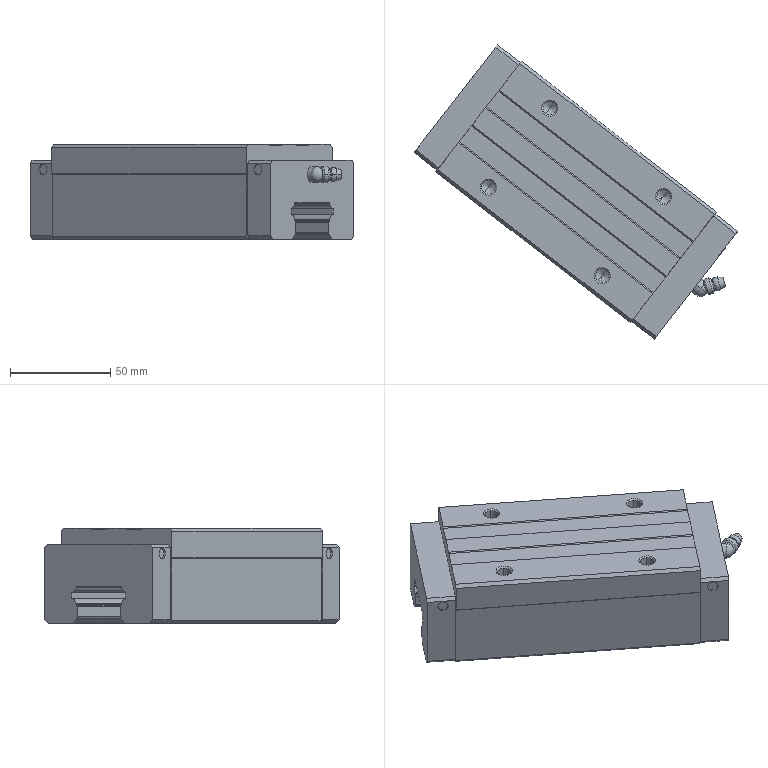Component | SolidWorks | 0803_101_Linear_Guide-1_0803_Z_Linear_Guide_2-1 | 1 solid | 122 faces | box 161.77 x 146.92 x 47.5 mm | volume 395212 mm3 | plane 53 | cylinder 38 | cone 20 | torus 8 | sphere 3 | commonest cylinder face diameters 6.8 x8 5.2 x8 5.719 x4 6.66 x2 8.1 x2 8 x2 2.021 x2 1.906 x2